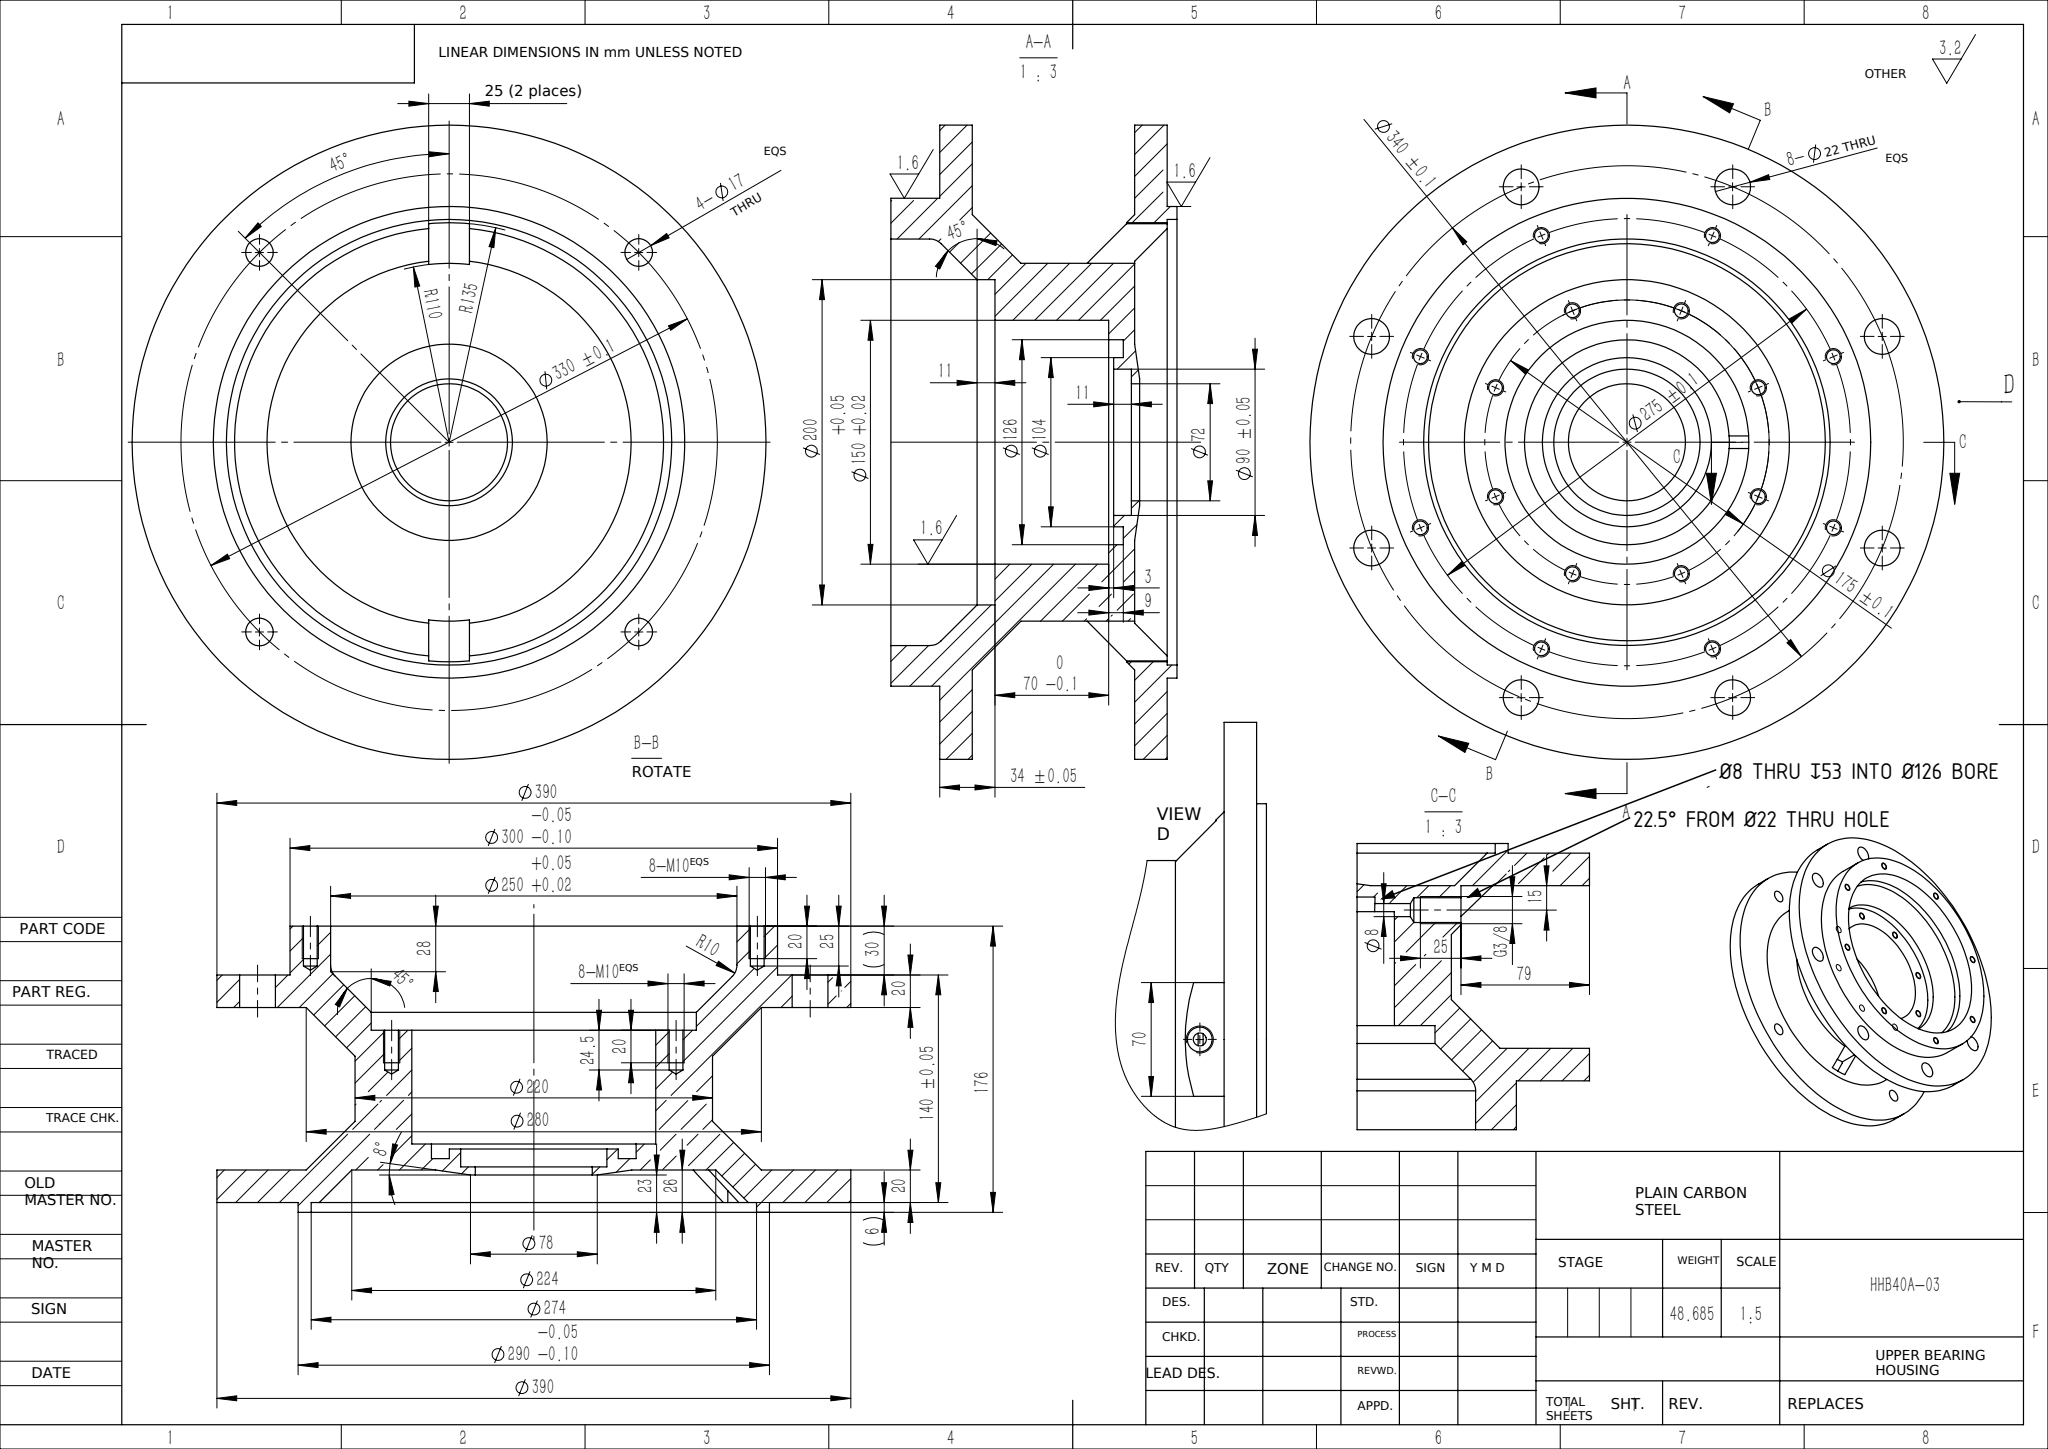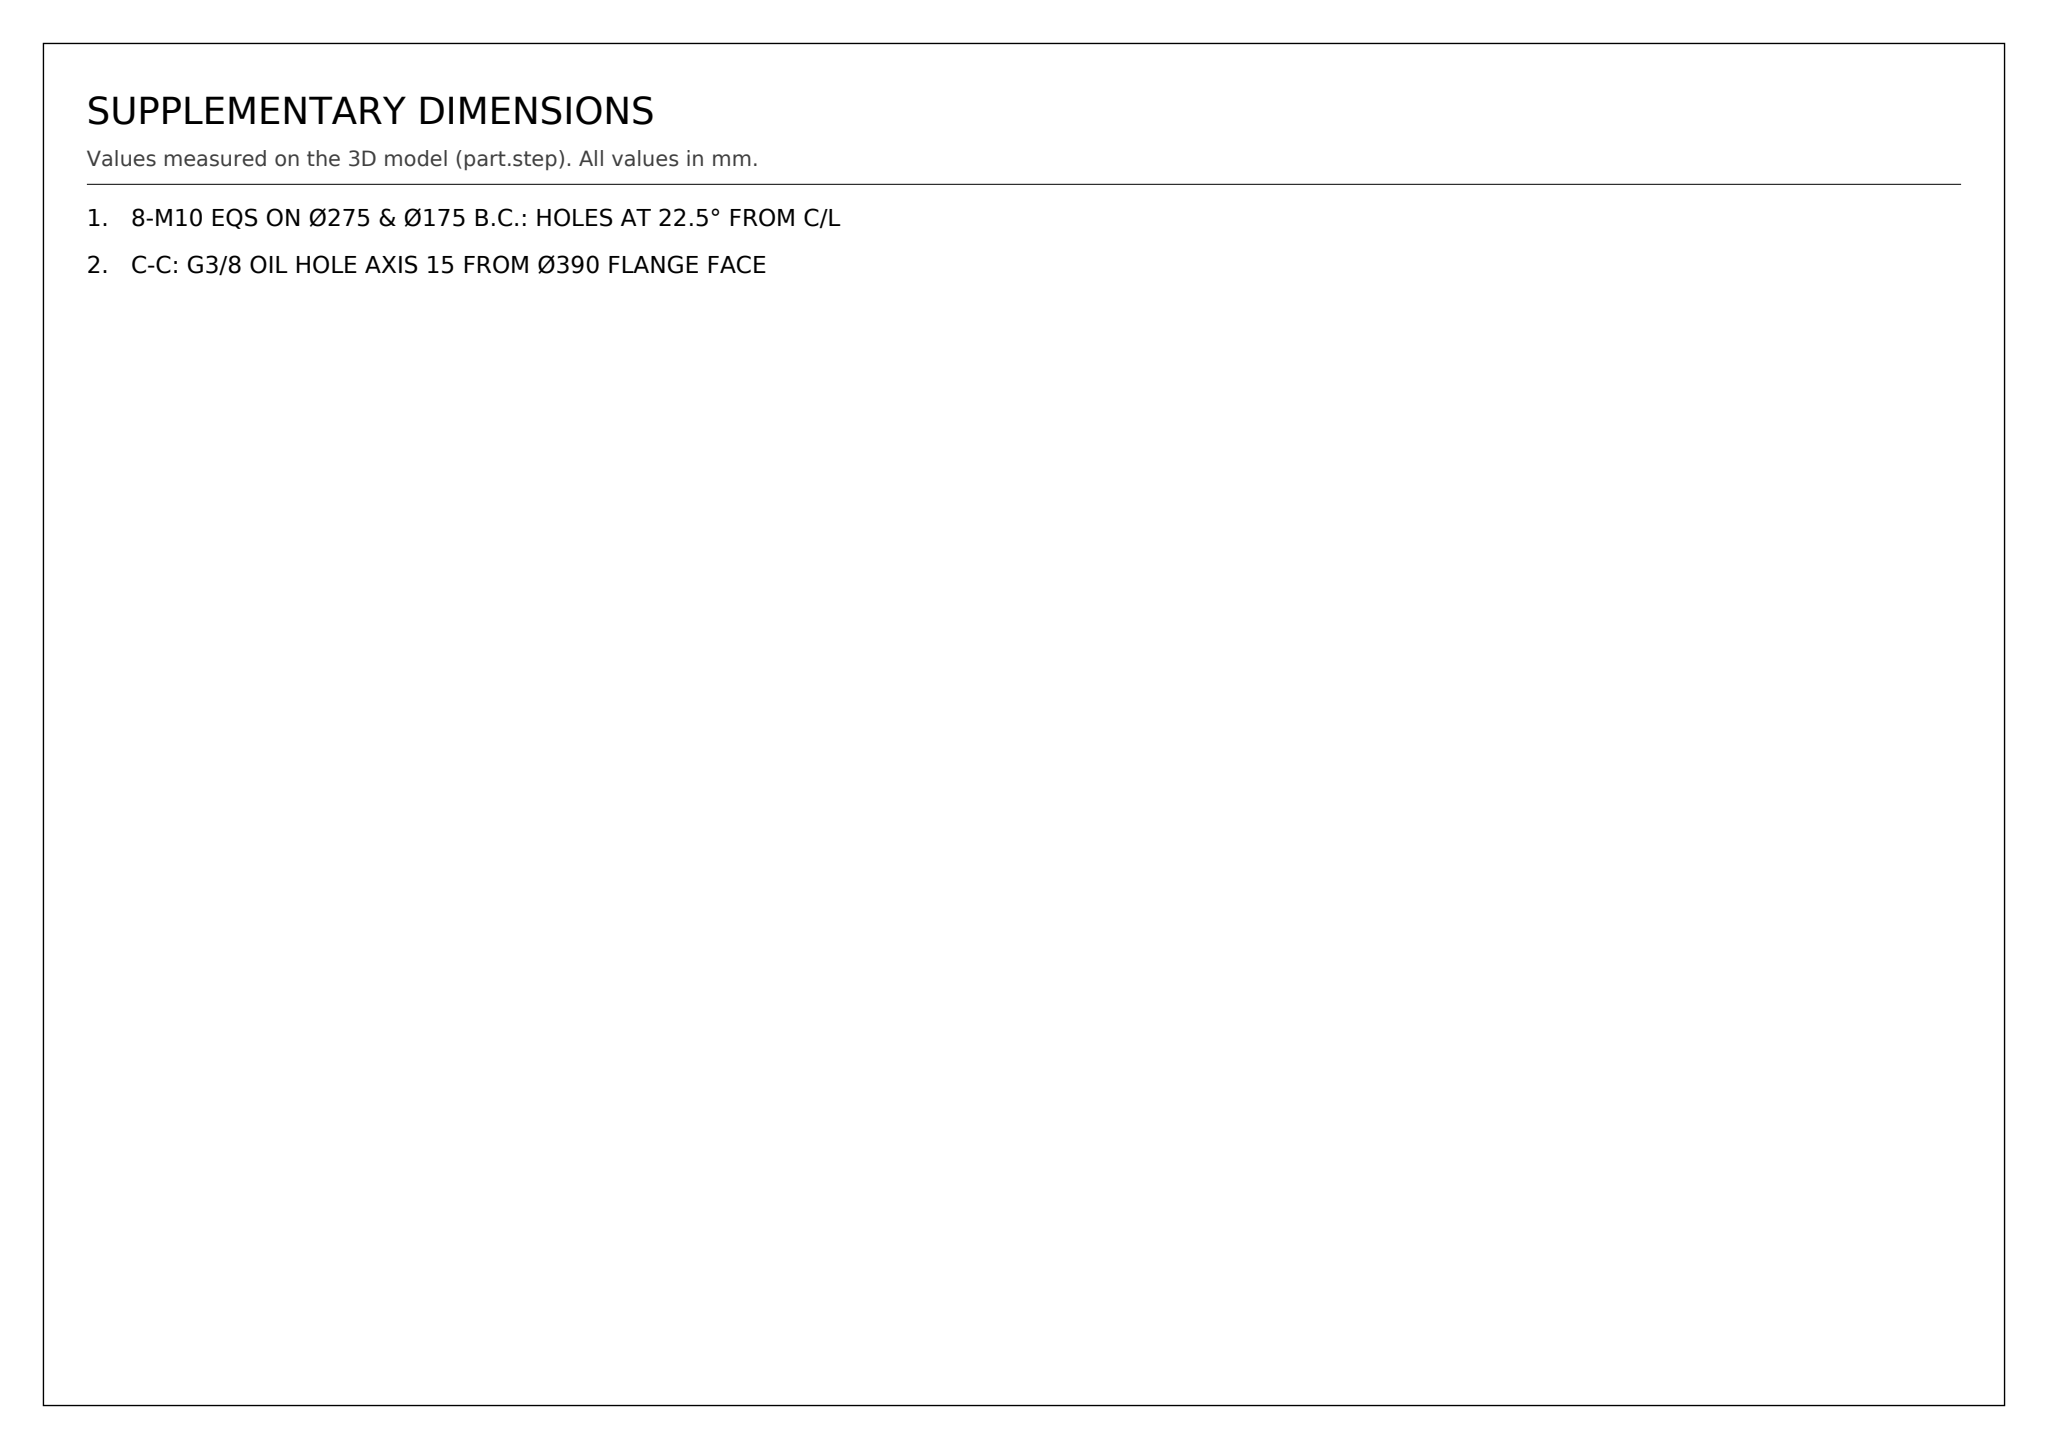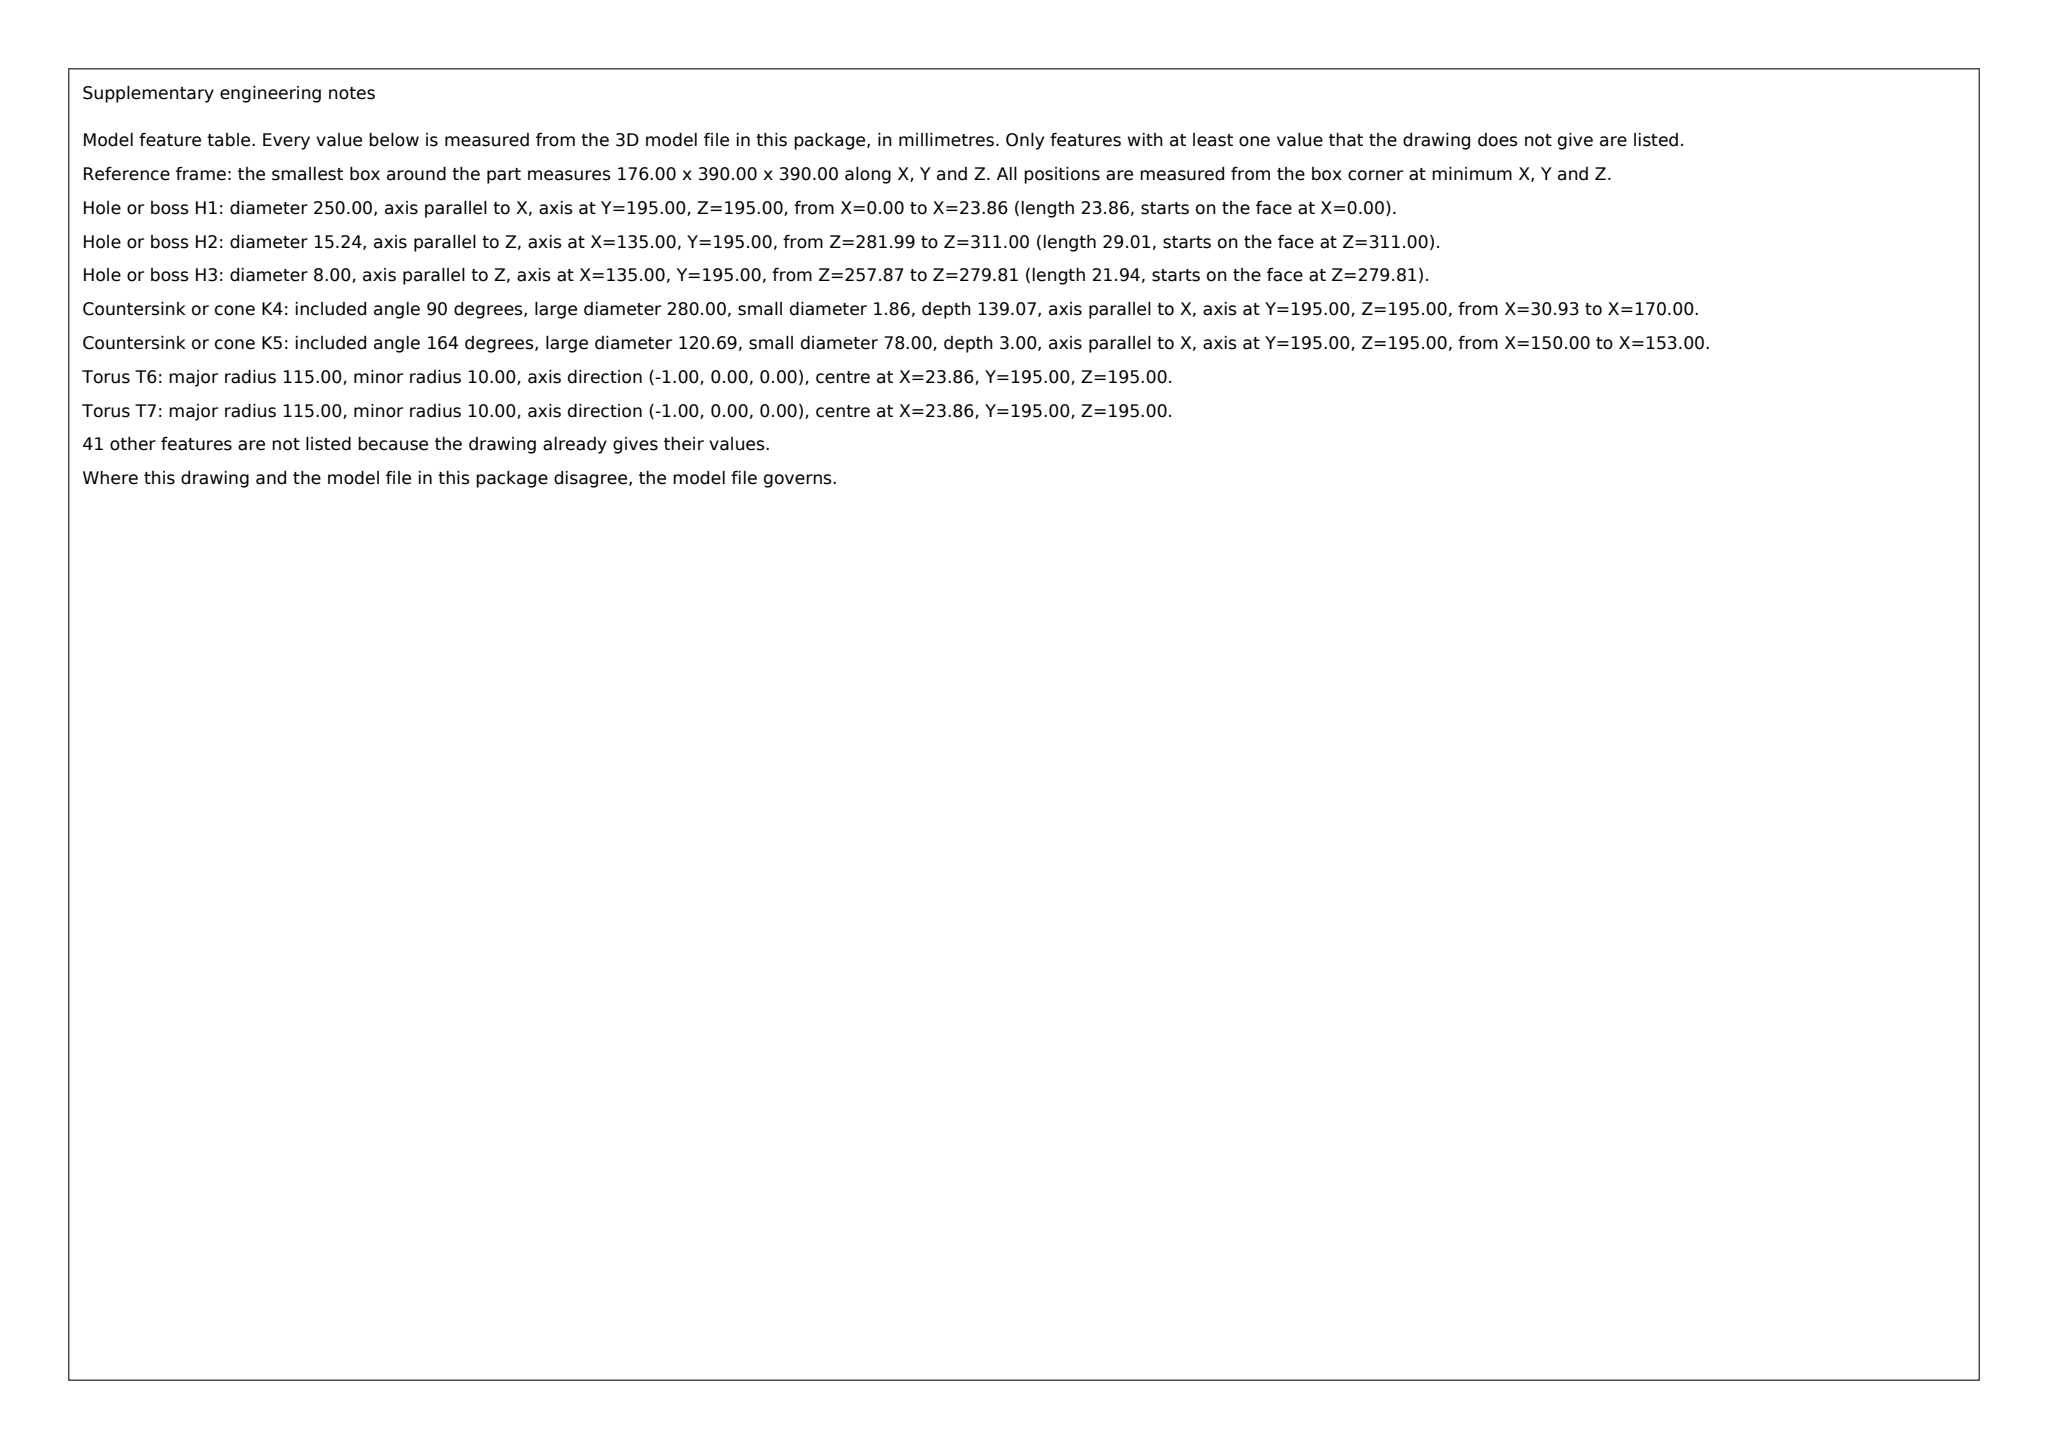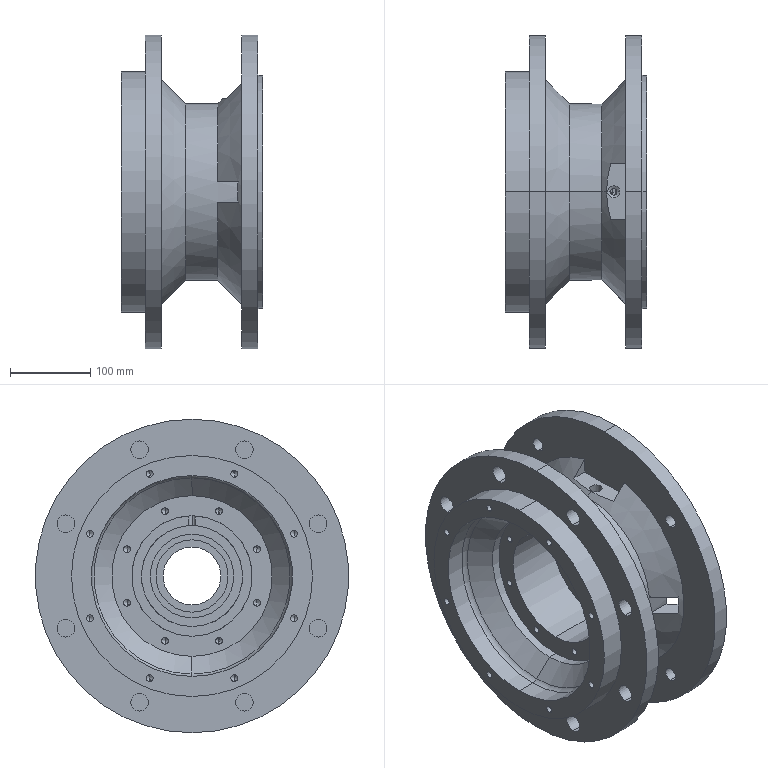Part | SolidWorks | mm | material PLAIN CARBON STEEL | 1 solid | 156 faces | box 176 x 390 x 390 mm | volume 6241663 mm3 | cylinder 88 | cone 45 | plane 21 | torus 2 | commonest cylinder face diameters 8.5 x32 22 x16 17 x8 390 x4 15.25 x2 8 x2 72 x2 90 x2
Drawing notes:
G3/8 oil port (section C-C) axis is radial, lying in the plane of the horizontal centerline (Y = axis centerline) at the notch flat: 22.5° from the nearest Ø22 THRU hole and 45° from the nearest Ø17 THRU hole; tap drill Ø15.25 from the Ø232 flat to R87, continuing Ø8 through to the bore. | from the solid: hole Ø15.25 axis z at [x135,y195] z282-311 and hole Ø8 axis z at [x135,y195] z257.9-279.8; Ø22 holes at y/z 129.9/352.1 etc (±22.5°), Ø17 holes at 311.7/311.7 etc (45°)
8-M10 EQS ON Ø275 & Ø175 B.C.: HOLES AT 22.5° FROM C/L | from the solid: M10 tap drills Ø8.5 at (142.4,322.0) r=137.5 and (114.2,161.5) r=87.5 from axis (195,195) = 22.5° off Y/Z centerlines
C-C: G3/8 OIL HOLE AXIS 15 FROM Ø390 FLANGE FACE | from the solid: Z-axis hole at x=135; Ø390 flange face plane at x=150 -> 150-135=15
Ø8 HOLE THRU INTO Ø126 BORE, DP 53 FROM G3/8 FLAT FACE | from the solid: Ø8 hole z=257.9-279.8 meets Ø126 bore at z=258; G3/8 Ø15.25 z=282-311, flat face plane z=311 -> 311-258=53
build123d program:
from build123d import *

# Parameters (mm, degrees)
CUT_EXTRUDE1_DEPTH      = 20
CUT_EXTRUDE2_DEPTH      = 38
CUT_EXTRUDE3_REACH      = 325.96
SKETCH4_R               = 8.5
CUT_EXTRUDE4_REACH      = 314.035
SKETCH5_R               = 11
CIRPATTERN1_COUNT       = 8
CIRPATTERN2_COUNT       = 8
CUT_EXTRUDE5_START      = 55
SKETCH10_R              = 4
CUT_EXTRUDE5_DEPTH      = 30
CUT_EXTRUDE6_START      = 116
SKETCH11_R              = 13
CUT_EXTRUDE6_DEPTH      = 212.148
G3_8_TAPPED_HOLE1_D     = 15.25
G3_8_TAPPED_HOLE1_DEPTH = 29.01
G3_8_TAPPED_HOLE1_TIP   = 4.582
SKETCH14_W              = 33.13
SKETCH14_H              = 70
CUT_EXTRUDE7_DEPTH      = 408.09


with BuildPart() as part:
    # Sketch1 → Revolve1 (revolve)
    with BuildSketch(Plane.XY, mode=Mode.PRIVATE) as revolve1_sk:
        with BuildLine():
            Line((0, 125), (23.858, 125))
            ThreePointArc((23.858, 125), (27.685, 124.239), (30.929, 122.071))
            Line((30.929, 122.071), (53, 100))
            Line((53, 100), (64, 100))
            Line((64, 100), (64, 75))
            Line((64, 75), (134, 75))
            Line((134, 75), (134, 63))
            Line((134, 63), (143, 63))
            Line((143, 63), (143, 52))
            Line((143, 52), (137, 52))
            Line((137, 52), (137, 45))
            Line((137, 45), (148, 45))
            Line((148, 45), (148, 36))
            Line((148, 36), (153, 36))
            Line((153, 36), (153, 39))
            Line((153, 39), (150, 60.346))
            Line((150, 60.346), (150, 112))
            Line((150, 112), (170, 132))
            Line((170, 132), (170, 137))
            Line((170, 137), (176, 137))
            Line((176, 137), (176, 145))
            Line((176, 145), (170, 145))
            Line((170, 145), (170, 195))
            Line((170, 195), (150, 195))
            Line((150, 195), (150, 140))
            Line((150, 140), (120, 110))
            Line((120, 110), (80, 110))
            Line((80, 110), (50, 140))
            Line((50, 140), (50, 195))
            Line((50, 195), (30, 195))
            Line((30, 195), (30, 150))
            Line((30, 150), (0, 150))
            Line((0, 150), (0, 125))
        make_face()
    revolve(revolve1_sk.sketch.rotate(Axis((0, 0, 0), (1, 0, 0)), 90), axis=Axis((0, 0, 0), (1, 0, 0)))

    # Sketch2 → Cut-Extrude1 (cut)
    with BuildSketch(Plane(origin=(170, 0, 0), x_dir=(0, 0, -1), z_dir=(1, 0, 0))):
        with BuildLine():
            Line((-12.5, 134.42), (-12.5, 99.216))
            ThreePointArc((-12.5, 99.216), (0, 100), (12.5, 99.216))
            Line((12.5, 99.216), (12.5, 134.42))
            ThreePointArc((12.5, 134.42), (0, 135), (-12.5, 134.42))
        make_face()
        with BuildLine():
            Line((12.5, -99.216), (12.5, -134.42))
            ThreePointArc((12.5, -134.42), (0, -135), (-12.5, -134.42))
            Line((-12.5, -134.42), (-12.5, -99.216))
            ThreePointArc((-12.5, -99.216), (0, -100), (12.5, -99.216))
        make_face()
    extrude(amount=-CUT_EXTRUDE1_DEPTH, mode=Mode.SUBTRACT)

    # Sketch3 → Cut-Extrude2 (cut)
    with BuildSketch(Plane(origin=(150, 0, 0), x_dir=(0, 0, -1), z_dir=(1, 0, 0))):
        with BuildLine():
            Line((12.5, -134.42), (12.5, -109.287))
            ThreePointArc((12.5, -109.287), (0, -110), (-12.5, -109.287))
            Line((-12.5, -109.287), (-12.5, -134.42))
            ThreePointArc((-12.5, -134.42), (0, -135), (12.5, -134.42))
        make_face()
        with BuildLine():
            Line((-12.5, 134.42), (-12.5, 109.287))
            ThreePointArc((-12.5, 109.287), (0, 110), (12.5, 109.287))
            Line((12.5, 109.287), (12.5, 134.42))
            ThreePointArc((12.5, 134.42), (0, 135), (-12.5, 134.42))
        make_face()
    extrude(amount=-CUT_EXTRUDE2_DEPTH, mode=Mode.SUBTRACT)

    # Sketch4 → Cut-Extrude3 (cut, up to next)
    with BuildSketch(Plane(origin=(170, 0, 0), x_dir=(0, 0, -1), z_dir=(1, 0, 0)), mode=Mode.PRIVATE) as cut_extrude3_sk1:
        with Locations((-116.673, 116.673)):
            Circle(SKETCH4_R)
    cut_extrude3_tool1 = extrude(cut_extrude3_sk1.sketch, amount=-CUT_EXTRUDE3_REACH, mode=Mode.PRIVATE) & part.part
    # Sketch4 → Cut-Extrude3 (cut, up to next)
    with BuildSketch(Plane(origin=(170, 0, 0), x_dir=(0, 0, -1), z_dir=(1, 0, 0)), mode=Mode.PRIVATE) as cut_extrude3_sk2:
        with Locations((116.673, 116.673)):
            Circle(SKETCH4_R)
    cut_extrude3_tool2 = extrude(cut_extrude3_sk2.sketch, amount=-CUT_EXTRUDE3_REACH, mode=Mode.PRIVATE) & part.part
    # Sketch4 → Cut-Extrude3 (cut, up to next)
    with BuildSketch(Plane(origin=(170, 0, 0), x_dir=(0, 0, -1), z_dir=(1, 0, 0)), mode=Mode.PRIVATE) as cut_extrude3_sk3:
        with Locations((116.673, -116.673)):
            Circle(SKETCH4_R)
    cut_extrude3_tool3 = extrude(cut_extrude3_sk3.sketch, amount=-CUT_EXTRUDE3_REACH, mode=Mode.PRIVATE) & part.part
    # Sketch4 → Cut-Extrude3 (cut, up to next)
    with BuildSketch(Plane(origin=(170, 0, 0), x_dir=(0, 0, -1), z_dir=(1, 0, 0)), mode=Mode.PRIVATE) as cut_extrude3_sk4:
        with Locations((-116.673, -116.673)):
            Circle(SKETCH4_R)
    cut_extrude3_tool4 = extrude(cut_extrude3_sk4.sketch, amount=-CUT_EXTRUDE3_REACH, mode=Mode.PRIVATE) & part.part
    add(cut_extrude3_tool1.solids().sort_by_distance((170, 116.673, 116.673))[0], mode=Mode.SUBTRACT)
    add(cut_extrude3_tool2.solids().sort_by_distance((170, 116.673, -116.673))[0], mode=Mode.SUBTRACT)
    add(cut_extrude3_tool3.solids().sort_by_distance((170, -116.673, -116.673))[0], mode=Mode.SUBTRACT)
    add(cut_extrude3_tool4.solids().sort_by_distance((170, -116.673, 116.673))[0], mode=Mode.SUBTRACT)

    # Sketch5 → Cut-Extrude4 (cut, up to next)
    with BuildSketch(Plane.ZY.offset(-30), mode=Mode.PRIVATE) as cut_extrude4_sk1:
        with Locations((-65.056, 157.06)):
            Circle(SKETCH5_R)
    cut_extrude4_tool1 = extrude(cut_extrude4_sk1.sketch, amount=-CUT_EXTRUDE4_REACH, mode=Mode.PRIVATE) & part.part
    # Sketch5 → Cut-Extrude4 (cut, up to next)
    with BuildSketch(Plane.ZY.offset(-30), mode=Mode.PRIVATE) as cut_extrude4_sk2:
        with Locations((65.056, 157.06)):
            Circle(SKETCH5_R)
    cut_extrude4_tool2 = extrude(cut_extrude4_sk2.sketch, amount=-CUT_EXTRUDE4_REACH, mode=Mode.PRIVATE) & part.part
    # Sketch5 → Cut-Extrude4 (cut, up to next)
    with BuildSketch(Plane.ZY.offset(-30), mode=Mode.PRIVATE) as cut_extrude4_sk3:
        with Locations((157.06, 65.056)):
            Circle(SKETCH5_R)
    cut_extrude4_tool3 = extrude(cut_extrude4_sk3.sketch, amount=-CUT_EXTRUDE4_REACH, mode=Mode.PRIVATE) & part.part
    # Sketch5 → Cut-Extrude4 (cut, up to next)
    with BuildSketch(Plane.ZY.offset(-30), mode=Mode.PRIVATE) as cut_extrude4_sk4:
        with Locations((157.06, -65.056)):
            Circle(SKETCH5_R)
    cut_extrude4_tool4 = extrude(cut_extrude4_sk4.sketch, amount=-CUT_EXTRUDE4_REACH, mode=Mode.PRIVATE) & part.part
    # Sketch5 → Cut-Extrude4 (cut, up to next)
    with BuildSketch(Plane.ZY.offset(-30), mode=Mode.PRIVATE) as cut_extrude4_sk5:
        with Locations((65.056, -157.06)):
            Circle(SKETCH5_R)
    cut_extrude4_tool5 = extrude(cut_extrude4_sk5.sketch, amount=-CUT_EXTRUDE4_REACH, mode=Mode.PRIVATE) & part.part
    # Sketch5 → Cut-Extrude4 (cut, up to next)
    with BuildSketch(Plane.ZY.offset(-30), mode=Mode.PRIVATE) as cut_extrude4_sk6:
        with Locations((-65.056, -157.06)):
            Circle(SKETCH5_R)
    cut_extrude4_tool6 = extrude(cut_extrude4_sk6.sketch, amount=-CUT_EXTRUDE4_REACH, mode=Mode.PRIVATE) & part.part
    # Sketch5 → Cut-Extrude4 (cut, up to next)
    with BuildSketch(Plane.ZY.offset(-30), mode=Mode.PRIVATE) as cut_extrude4_sk7:
        with Locations((-157.06, -65.056)):
            Circle(SKETCH5_R)
    cut_extrude4_tool7 = extrude(cut_extrude4_sk7.sketch, amount=-CUT_EXTRUDE4_REACH, mode=Mode.PRIVATE) & part.part
    # Sketch5 → Cut-Extrude4 (cut, up to next)
    with BuildSketch(Plane.ZY.offset(-30), mode=Mode.PRIVATE) as cut_extrude4_sk8:
        with Locations((-157.06, 65.056)):
            Circle(SKETCH5_R)
    cut_extrude4_tool8 = extrude(cut_extrude4_sk8.sketch, amount=-CUT_EXTRUDE4_REACH, mode=Mode.PRIVATE) & part.part
    add(cut_extrude4_tool1.solids().sort_by_distance((30, 157.06, -65.056))[0], mode=Mode.SUBTRACT)
    add(cut_extrude4_tool2.solids().sort_by_distance((30, 157.06, 65.056))[0], mode=Mode.SUBTRACT)
    add(cut_extrude4_tool3.solids().sort_by_distance((30, 65.056, 157.06))[0], mode=Mode.SUBTRACT)
    add(cut_extrude4_tool4.solids().sort_by_distance((30, -65.056, 157.06))[0], mode=Mode.SUBTRACT)
    add(cut_extrude4_tool5.solids().sort_by_distance((30, -157.06, 65.056))[0], mode=Mode.SUBTRACT)
    add(cut_extrude4_tool6.solids().sort_by_distance((30, -157.06, -65.056))[0], mode=Mode.SUBTRACT)
    add(cut_extrude4_tool7.solids().sort_by_distance((30, -65.056, -157.06))[0], mode=Mode.SUBTRACT)
    add(cut_extrude4_tool8.solids().sort_by_distance((30, 65.056, -157.06))[0], mode=Mode.SUBTRACT)

    # Sketch7 → M10 Tapped Hole1 (revolve, cut)
    with BuildSketch(Plane(origin=(0, 127.033, -52.619), x_dir=(0, 0, 1), z_dir=(0, 1, 0))):
        Polygon((0, 0), (0, 27.054), (4.25, 24.5), (4.25, 0), align=None)
    m10_tapped_hole1 = revolve(axis=Axis((-6.35, 127.033, -52.619), (1, 0, 0)), mode=Mode.SUBTRACT)

    # CirPattern1: M10 Tapped Hole1 ×8 about axis
    cirpattern1_axis = Axis((0, 0, 0), (1, 0, 0))
    for i in range(1, CIRPATTERN1_COUNT):
        add(m10_tapped_hole1.rotate(cirpattern1_axis, i * 360 / CIRPATTERN1_COUNT), mode=Mode.SUBTRACT)

    # Sketch9 → M10 Tapped Hole2 (revolve, cut)
    with BuildSketch(Plane(origin=(64, 80.839, -33.485), x_dir=(0, 0, 1), z_dir=(0, 1, 0))):
        Polygon((0, 0), (0, 27.054), (4.25, 24.5), (4.25, 0), align=None)
    m10_tapped_hole2 = revolve(axis=Axis((57.65, 80.839, -33.485), (1, 0, 0)), mode=Mode.SUBTRACT)

    # CirPattern2: M10 Tapped Hole2 ×8 about axis
    cirpattern2_axis = Axis((0, 0, 0), (1, 0, 0))
    for i in range(1, CIRPATTERN2_COUNT):
        add(m10_tapped_hole2.rotate(cirpattern2_axis, i * 360 / CIRPATTERN2_COUNT), mode=Mode.SUBTRACT)

    # Sketch10 → Cut-Extrude5 (cut)
    with BuildSketch(Plane.XY.offset(CUT_EXTRUDE5_START)):
        with Locations((135, 0)):
            Circle(SKETCH10_R)
    extrude(amount=CUT_EXTRUDE5_DEPTH, mode=Mode.SUBTRACT)

    # Sketch11 → Cut-Extrude6 (cut, through all)
    with BuildSketch(Plane.XY.offset(CUT_EXTRUDE6_START)):
        with Locations((135, 0)):
            Circle(SKETCH11_R)
    extrude(amount=CUT_EXTRUDE6_DEPTH, mode=Mode.SUBTRACT)

    # G3_8 Tapped Hole1
    with Locations(Plane(origin=(135, 0, 116), x_dir=(1, 0, 0), z_dir=(0, 0, 1))):
        with Locations((0, 0)):
            Hole(G3_8_TAPPED_HOLE1_D / 2, depth=G3_8_TAPPED_HOLE1_DEPTH)
            with Locations((0, 0, -(G3_8_TAPPED_HOLE1_DEPTH + G3_8_TAPPED_HOLE1_TIP / 2))):  # 118° drill point
                Cone(0, G3_8_TAPPED_HOLE1_D / 2, G3_8_TAPPED_HOLE1_TIP, mode=Mode.SUBTRACT)

    # Sketch14 → Cut-Extrude7 (cut, through all)
    with BuildSketch(Plane.XY.offset(116)):
        with Locations((133.435, 0)):
            Rectangle(SKETCH14_W, SKETCH14_H)
    extrude(amount=CUT_EXTRUDE7_DEPTH, mode=Mode.SUBTRACT)


solid = part.part